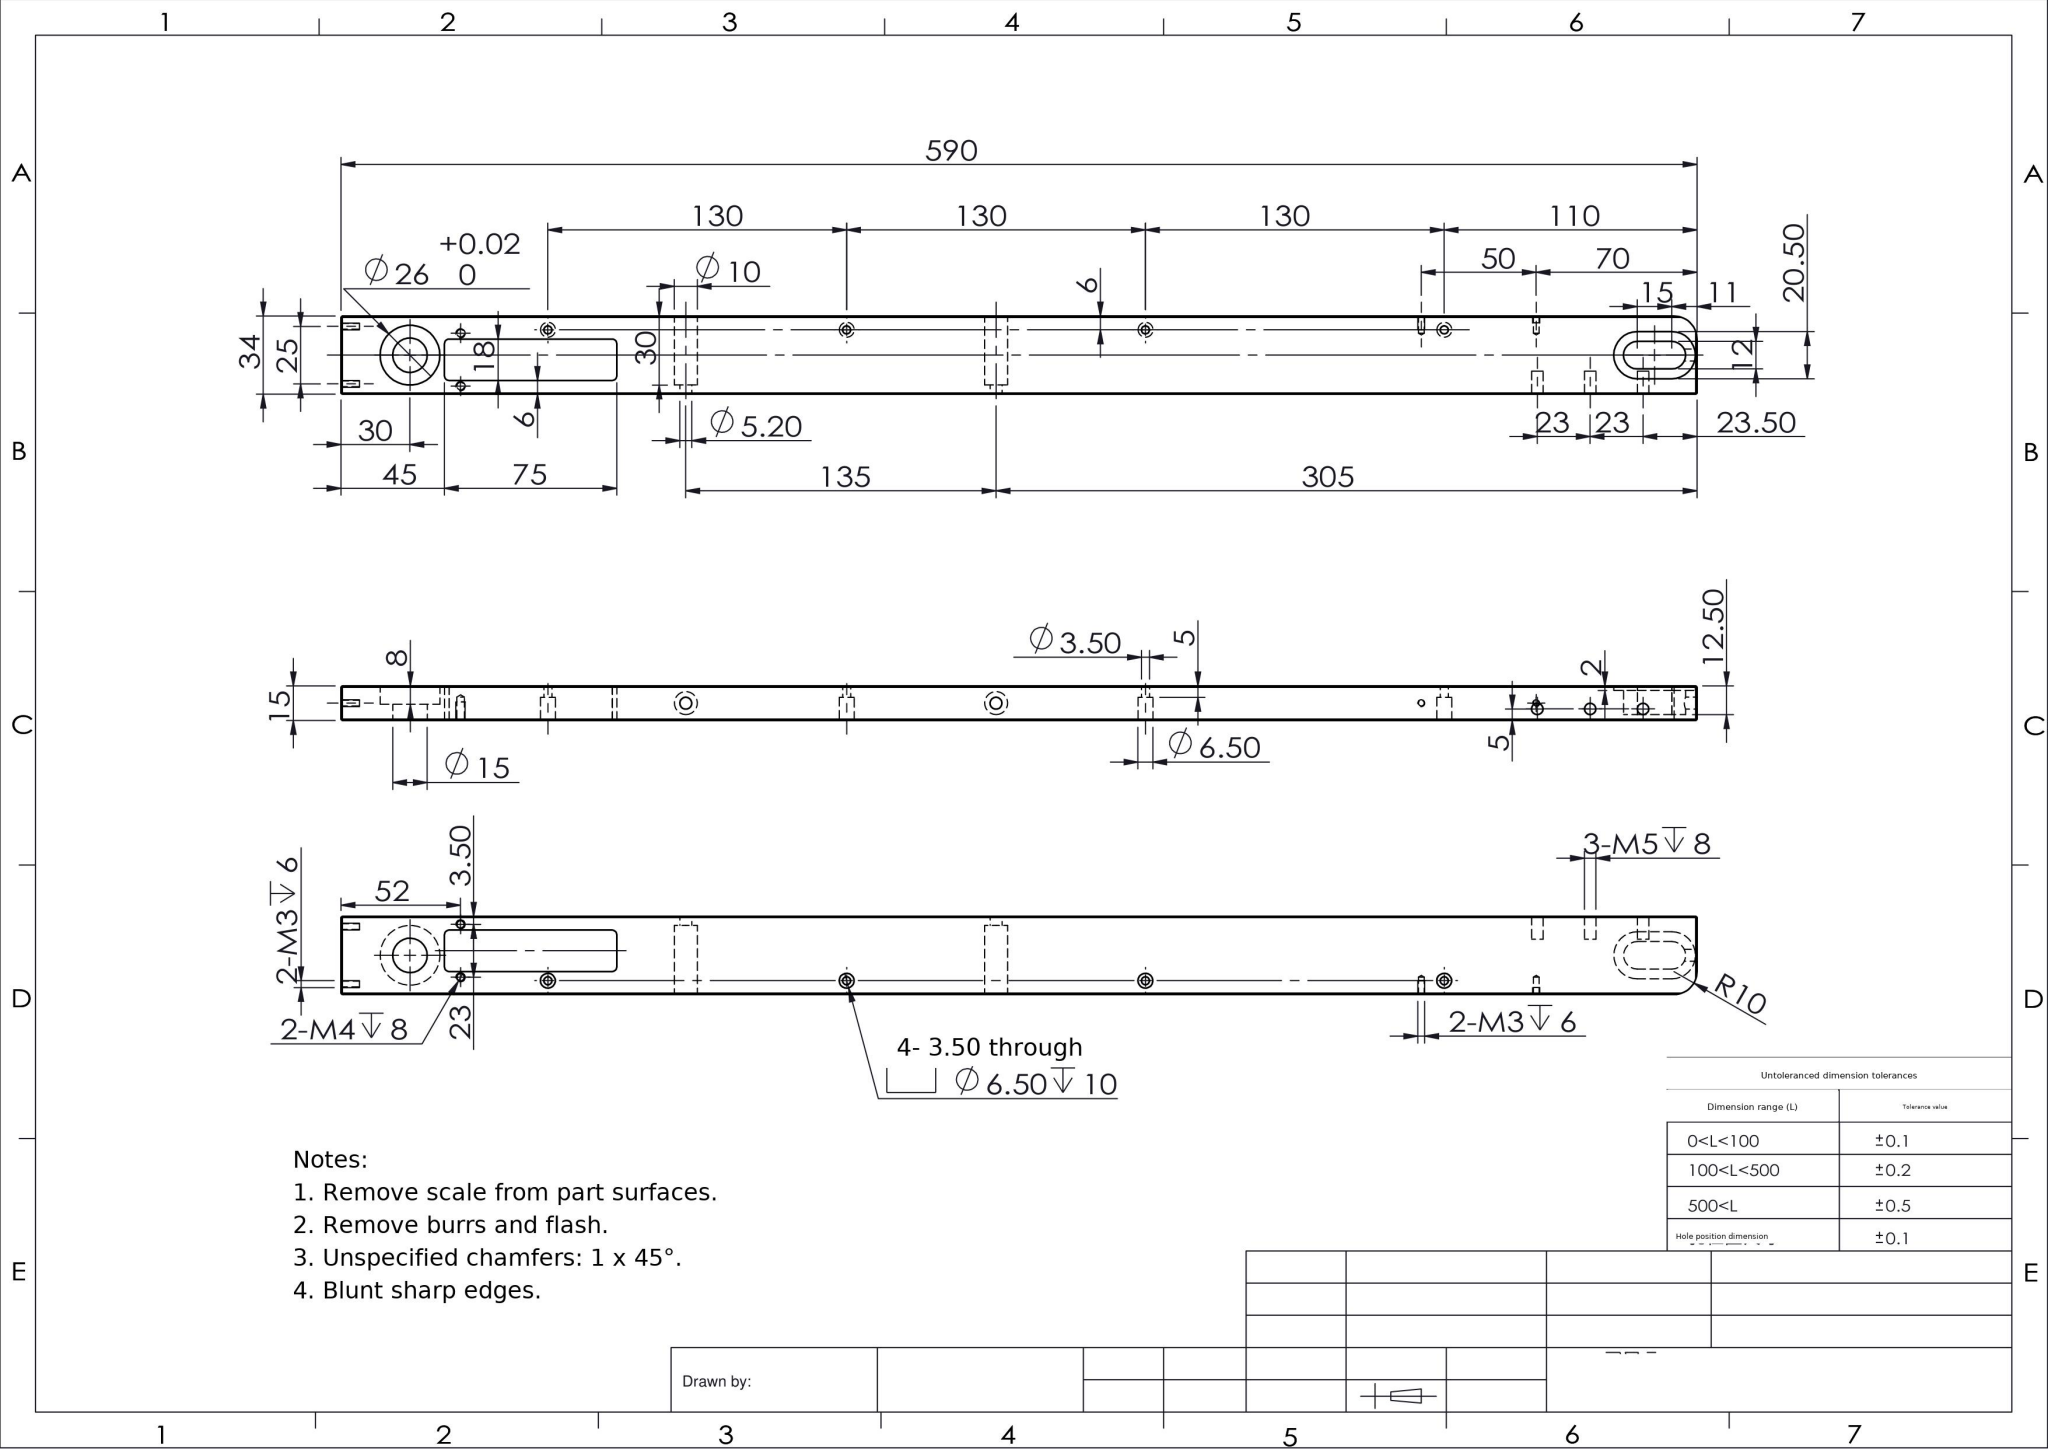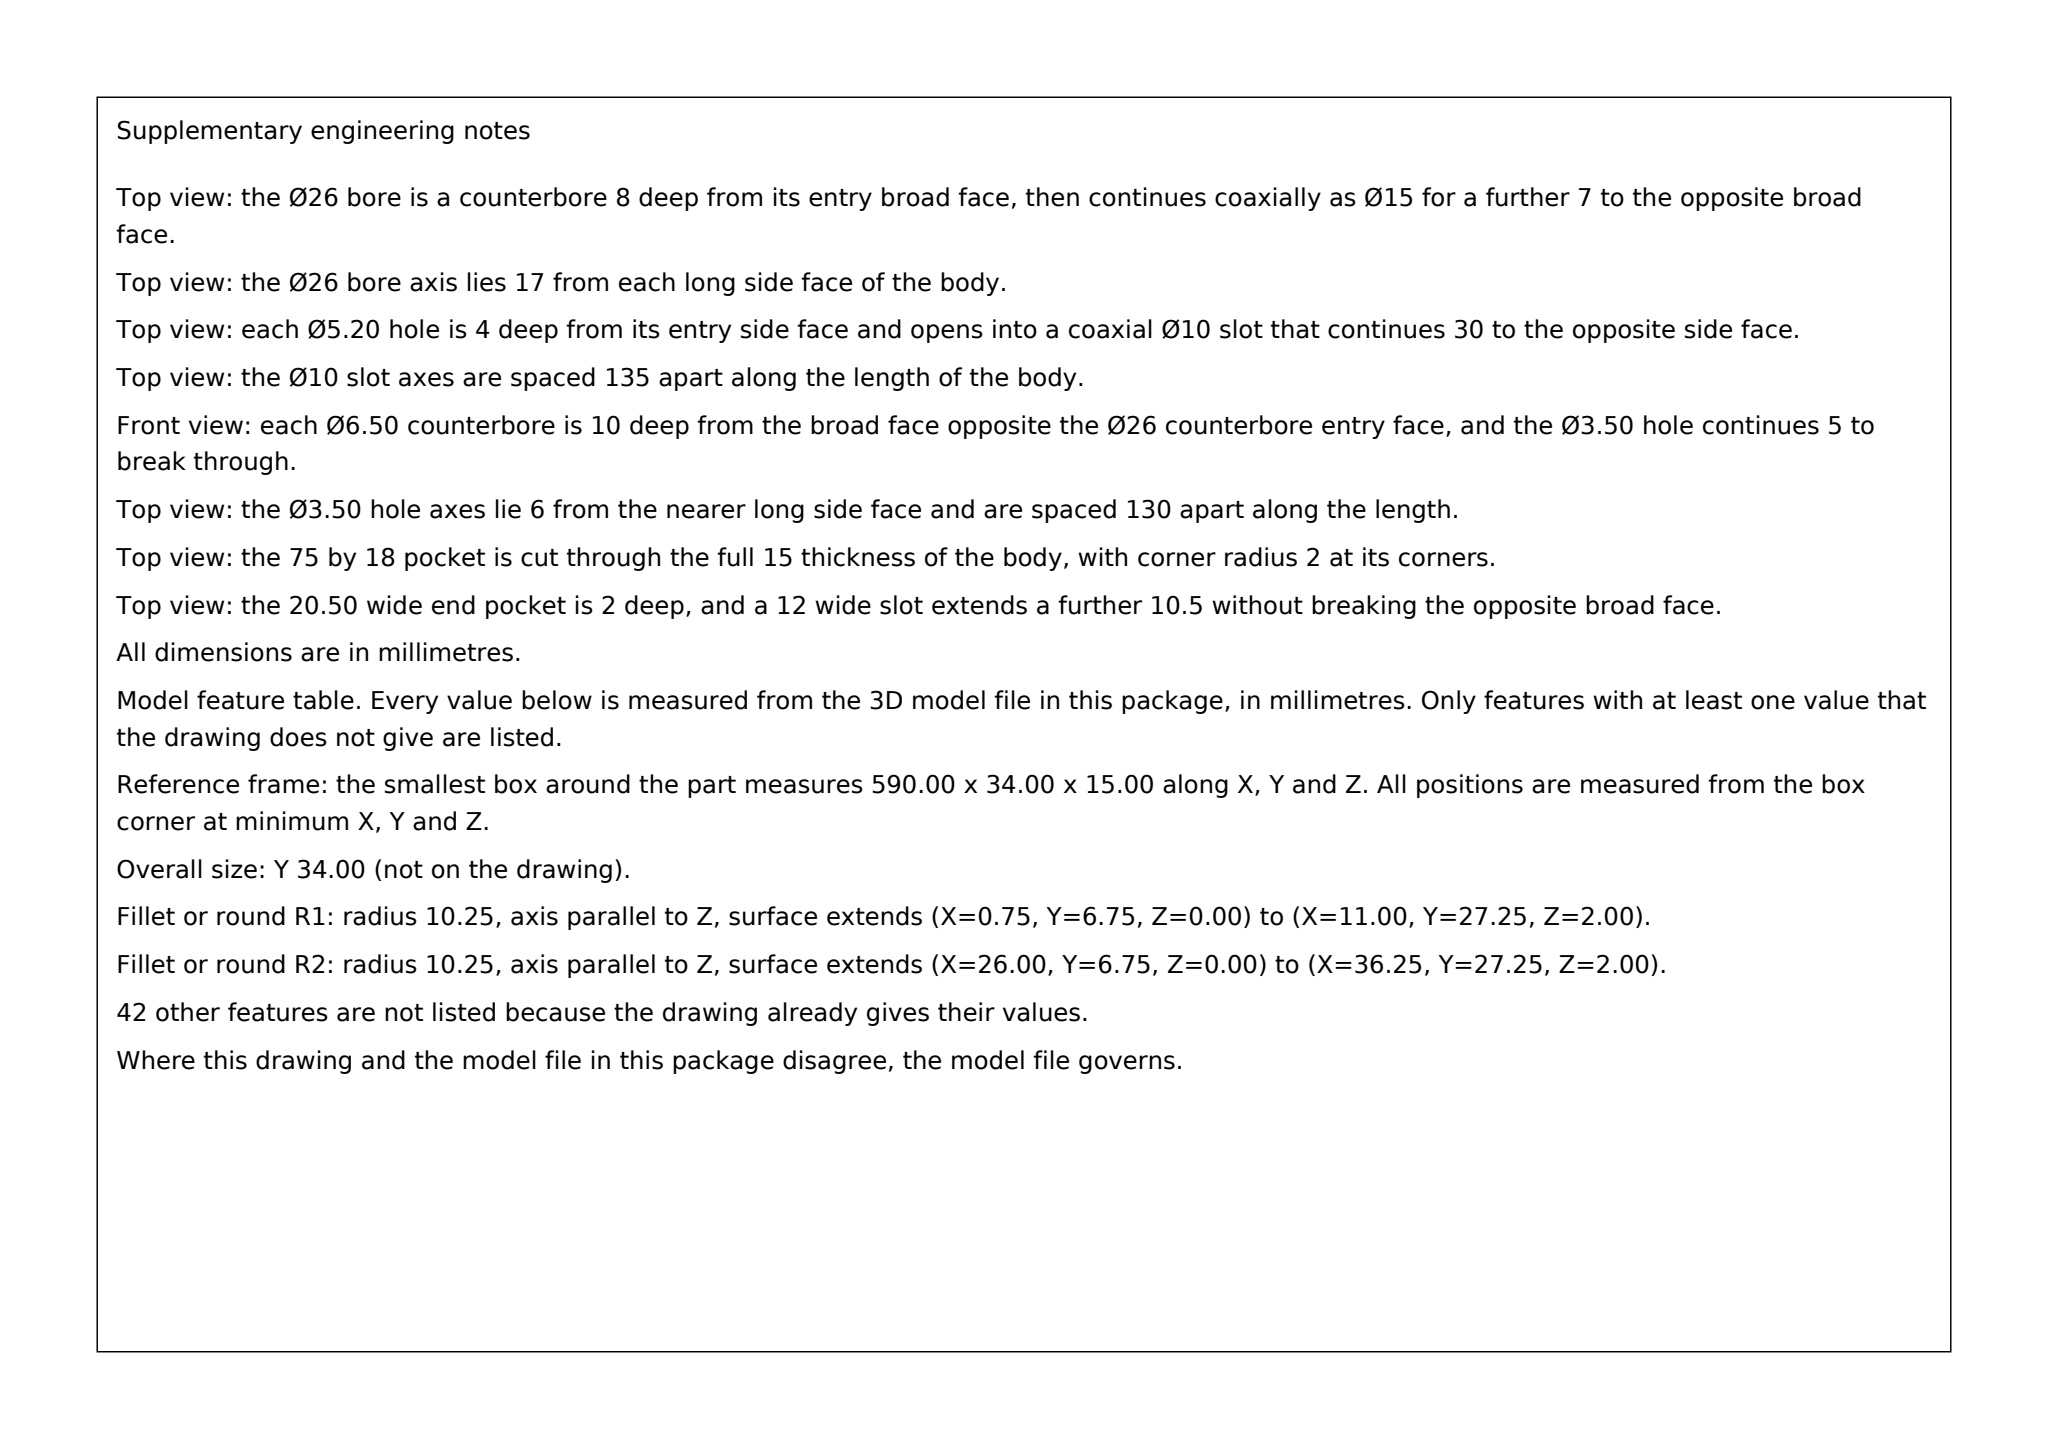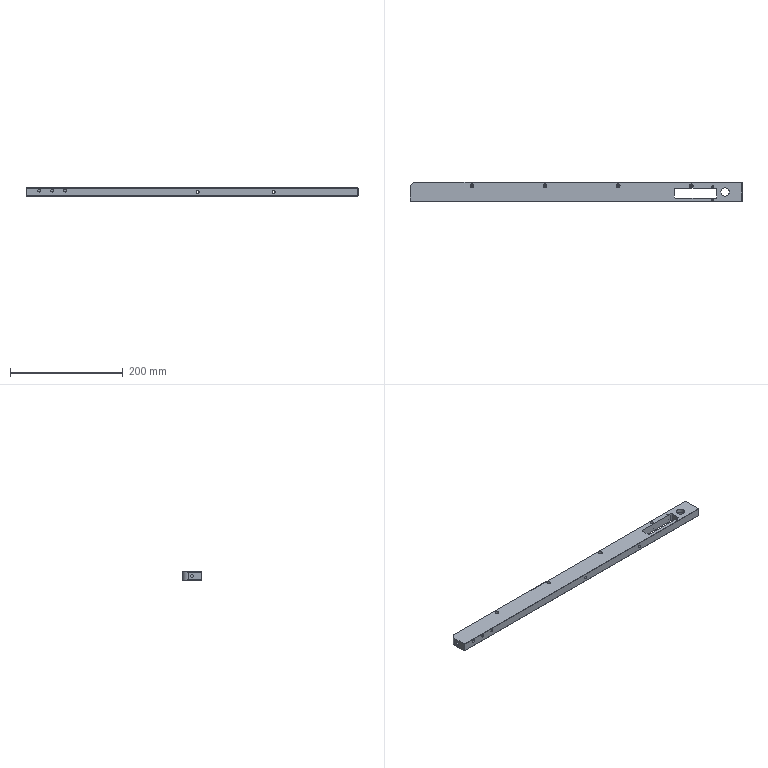Part | SolidWorks | mm | 1 solid | 112 faces | box 590 x 34 x 15 mm | volume 262796 mm3 | cylinder 59 | plane 45 | cone 8 | commonest cylinder face diameters 2.5 x8 6.5 x8 3.5 x8 5.2 x6 5 x6 10 x4 3.3 x4 4 x4
Drawing notes:
4X Ø4 THRU AT 75x18 SLOT CORNERS, C/L 2 IN FROM SLOT EDGES | from the solid: Ø4.0 z-axis cyls, L=15 (full 15 thk), at (472,8),(472,22),(543,8),(543,22); slot bounded by x-planes 470/545 and y 6/24 -> centers inset 2 from each slot edge (= 47 & 118 from LH end, y 8 & 22)
Ø5.20 DP 5.59 BLIND IN END FACE (R10 END), ON C/L 17 & 7.5 | from the solid: Ø5.2 x-axis cyl, pos y=17, z=7.5, length 5.59, starting at end face x-plane 0 (R10/obround end); no breakout into Ø12 obround at x=11/26